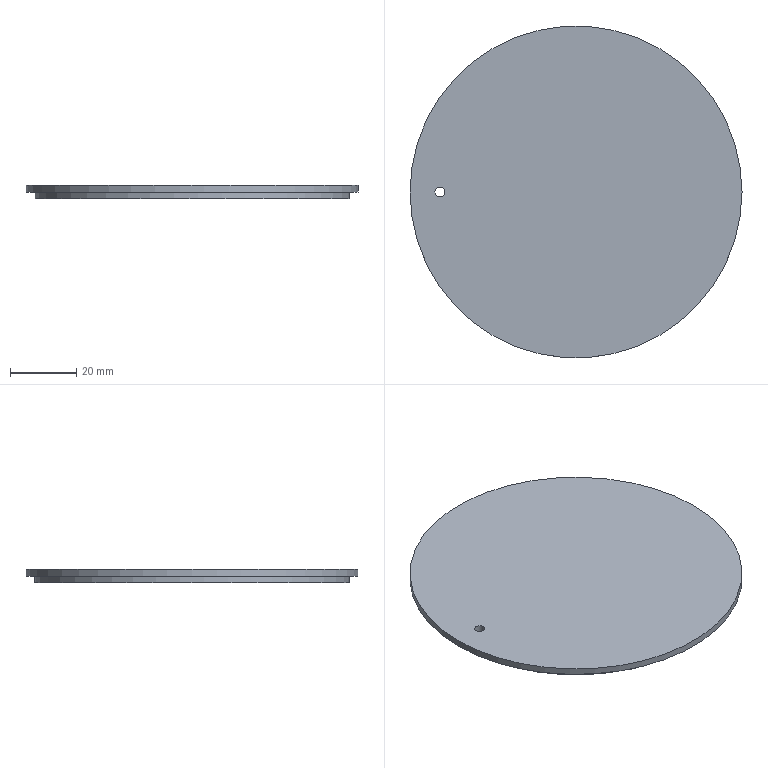Component | NX | BASE_COVER | 1 solid | 6 faces | box 100 x 100 x 4 mm | volume 29796 mm3 | cylinder 3 | plane 3 | commonest cylinder face diameters 94.8 x1 100 x1 3 x1
STEP:
#1=CARTESIAN_POINT('',(0.,0.,0.));
#2=DIRECTION('',(0.,0.,1.));
#3=DIRECTION('',(1.,0.,0.));
#4=AXIS2_PLACEMENT_3D('',#1,#2,#3);
#5=CARTESIAN_POINT('',(45.896,-15.585,-0.4905));
#6=VERTEX_POINT('',#5);
#7=CARTESIAN_POINT('',(-1.504,-15.585,-0.4905));
#8=DIRECTION('',(0.,0.,-1.));
#9=DIRECTION('',(1.,0.,0.));
#10=AXIS2_PLACEMENT_3D('',#7,#8,#9);
#11=CIRCLE('',#10,47.4);
#12=CARTESIAN_POINT('',(-1.504,-15.585,-0.4905));
#13=DIRECTION('',(0.,0.,-1.));
#14=DIRECTION('',(1.,0.,0.));
#15=AXIS2_PLACEMENT_3D('',#12,#13,#14);
#16=CYLINDRICAL_SURFACE('',#15,47.4);
#17=CARTESIAN_POINT('',(0.,0.));
#18=DIRECTION('',(1.,0.));
#19=VECTOR('',#18,1.);
#20=LINE('',#17,#19);
#21=(GEOMETRIC_REPRESENTATION_CONTEXT(2)PARAMETRIC_REPRESENTATION_CONTEXT()REPRESENTATION_CONTEXT('',''));
#22=DEFINITIONAL_REPRESENTATION('',(#20),#21);
#23=PCURVE('',#16,#22);
#24=CARTESIAN_POINT('',(-1.504,-15.585,-0.4905));
#25=DIRECTION('',(0.,0.,-1.));
#26=DIRECTION('',(1.,0.,0.));
#27=AXIS2_PLACEMENT_3D('',#24,#25,#26);
#28=PLANE('',#27);
#29=CARTESIAN_POINT('',(0.,0.));
#30=DIRECTION('',(1.,0.));
#31=AXIS2_PLACEMENT_2D('',#29,#30);
#32=CIRCLE('',#31,47.4);
#33=(GEOMETRIC_REPRESENTATION_CONTEXT(2)PARAMETRIC_REPRESENTATION_CONTEXT()REPRESENTATION_CONTEXT('',''));
#34=DEFINITIONAL_REPRESENTATION('',(#32),#33);
#35=PCURVE('',#28,#34);
#36=SURFACE_CURVE('',#11,(#23,#35),.PCURVE_S1.);
#37=EDGE_CURVE('',#6,#6,#36,.T.);
#38=ORIENTED_EDGE('',*,*,#37,.T.);
#39=CARTESIAN_POINT('',(45.896,-15.585,-2.49));
#40=VERTEX_POINT('',#39);
#41=CARTESIAN_POINT('',(45.896,-15.585,-0.4905));
#42=CARTESIAN_POINT('',(45.896,-15.585,-2.49));
#43=B_SPLINE_CURVE_WITH_KNOTS('',1,(#41,#42),.UNSPECIFIED.,.F.,.F.,(2,2),(0.,2.),.PIECEWISE_BEZIER_KNOTS.);
#44=CARTESIAN_POINT('',(6.283,0.));
#45=DIRECTION('',(0.,1.));
#46=VECTOR('',#45,1.);
#47=LINE('',#44,#46);
#48=(GEOMETRIC_REPRESENTATION_CONTEXT(2)PARAMETRIC_REPRESENTATION_CONTEXT()REPRESENTATION_CONTEXT('',''));
#49=DEFINITIONAL_REPRESENTATION('',(#47),#48);
#50=PCURVE('',#16,#49);
#51=CARTESIAN_POINT('',(0.,0.));
#52=DIRECTION('',(0.,1.));
#53=VECTOR('',#52,1.);
#54=LINE('',#51,#53);
#55=(GEOMETRIC_REPRESENTATION_CONTEXT(2)PARAMETRIC_REPRESENTATION_CONTEXT()REPRESENTATION_CONTEXT('',''));
#56=DEFINITIONAL_REPRESENTATION('',(#54),#55);
#57=PCURVE('',#16,#56);
#58=SEAM_CURVE('',#43,(#50,#57),.PCURVE_S1.);
#59=EDGE_CURVE('',#6,#40,#58,.T.);
#60=ORIENTED_EDGE('',*,*,#59,.T.);
#61=CARTESIAN_POINT('',(-1.504,-15.585,-2.49));
#62=DIRECTION('',(0.,0.,-1.));
#63=DIRECTION('',(1.,0.,0.));
#64=AXIS2_PLACEMENT_3D('',#61,#62,#63);
#65=CIRCLE('',#64,47.4);
#66=CARTESIAN_POINT('',(0.,2.));
#67=DIRECTION('',(1.,0.));
#68=VECTOR('',#67,1.);
#69=LINE('',#66,#68);
#70=(GEOMETRIC_REPRESENTATION_CONTEXT(2)PARAMETRIC_REPRESENTATION_CONTEXT()REPRESENTATION_CONTEXT('',''));
#71=DEFINITIONAL_REPRESENTATION('',(#69),#70);
#72=PCURVE('',#16,#71);
#73=CARTESIAN_POINT('',(-1.504,-15.585,-2.49));
#74=DIRECTION('',(0.,0.,-1.));
#75=DIRECTION('',(1.,0.,0.));
#76=AXIS2_PLACEMENT_3D('',#73,#74,#75);
#77=PLANE('',#76);
#78=CARTESIAN_POINT('',(0.,0.));
#79=DIRECTION('',(1.,0.));
#80=AXIS2_PLACEMENT_2D('',#78,#79);
#81=CIRCLE('',#80,47.4);
#82=(GEOMETRIC_REPRESENTATION_CONTEXT(2)PARAMETRIC_REPRESENTATION_CONTEXT()REPRESENTATION_CONTEXT('',''));
#83=DEFINITIONAL_REPRESENTATION('',(#81),#82);
#84=PCURVE('',#77,#83);
#85=SURFACE_CURVE('',#65,(#72,#84),.PCURVE_S1.);
#86=EDGE_CURVE('',#40,#40,#85,.T.);
#87=ORIENTED_EDGE('',*,*,#86,.F.);
#88=ORIENTED_EDGE('',*,*,#59,.F.);
#89=EDGE_LOOP('',(#38,#60,#87,#88));
#90=FACE_BOUND('',#89,.T.);
#91=ADVANCED_FACE('',(#90),#16,.T.);
#92=CARTESIAN_POINT('',(-41.004,-15.585,-2.49));
#93=VERTEX_POINT('',#92);
#94=CARTESIAN_POINT('',(-42.504,-15.585,-2.49));
#95=DIRECTION('',(0.,0.,-1.));
#96=DIRECTION('',(1.,0.,0.));
#97=AXIS2_PLACEMENT_3D('',#94,#95,#96);
#98=CIRCLE('',#97,1.5);
#99=CARTESIAN_POINT('',(-41.,0.));
#100=DIRECTION('',(1.,0.));
#101=AXIS2_PLACEMENT_2D('',#99,#100);
#102=CIRCLE('',#101,1.5);
#103=(GEOMETRIC_REPRESENTATION_CONTEXT(2)PARAMETRIC_REPRESENTATION_CONTEXT()REPRESENTATION_CONTEXT('',''));
#104=DEFINITIONAL_REPRESENTATION('',(#102),#103);
#105=PCURVE('',#77,#104);
#106=CARTESIAN_POINT('',(-42.504,-15.585,8.01));
#107=DIRECTION('',(0.,0.,-1.));
#108=DIRECTION('',(1.,0.,0.));
#109=AXIS2_PLACEMENT_3D('',#106,#107,#108);
#110=CYLINDRICAL_SURFACE('',#109,1.5);
#111=CARTESIAN_POINT('',(0.,10.5));
#112=DIRECTION('',(1.,0.));
#113=VECTOR('',#112,1.);
#114=LINE('',#111,#113);
#115=(GEOMETRIC_REPRESENTATION_CONTEXT(2)PARAMETRIC_REPRESENTATION_CONTEXT()REPRESENTATION_CONTEXT('',''));
#116=DEFINITIONAL_REPRESENTATION('',(#114),#115);
#117=PCURVE('',#110,#116);
#118=SURFACE_CURVE('',#98,(#105,#117),.PCURVE_S1.);
#119=EDGE_CURVE('',#93,#93,#118,.T.);
#120=ORIENTED_EDGE('',*,*,#119,.F.);
#121=EDGE_LOOP('',(#120));
#122=FACE_BOUND('',#121,.T.);
#123=ORIENTED_EDGE('',*,*,#86,.T.);
#124=EDGE_LOOP('',(#123));
#125=FACE_BOUND('',#124,.T.);
#126=ADVANCED_FACE('',(#122,#125),#77,.T.);
#127=CARTESIAN_POINT('',(48.496,-15.585,-0.4905));
#128=VERTEX_POINT('',#127);
#129=CARTESIAN_POINT('',(-1.504,-15.585,-0.4905));
#130=DIRECTION('',(0.,0.,-1.));
#131=DIRECTION('',(1.,0.,0.));
#132=AXIS2_PLACEMENT_3D('',#129,#130,#131);
#133=CIRCLE('',#132,50.);
#134=CARTESIAN_POINT('',(-1.504,-15.585,-0.4905));
#135=DIRECTION('',(0.,0.,1.));
#136=DIRECTION('',(-1.,0.,0.));
#137=AXIS2_PLACEMENT_3D('',#134,#135,#136);
#138=CYLINDRICAL_SURFACE('',#137,50.);
#139=CARTESIAN_POINT('',(9.425,0.));
#140=DIRECTION('',(-1.,0.));
#141=VECTOR('',#140,1.);
#142=LINE('',#139,#141);
#143=(GEOMETRIC_REPRESENTATION_CONTEXT(2)PARAMETRIC_REPRESENTATION_CONTEXT()REPRESENTATION_CONTEXT('',''));
#144=DEFINITIONAL_REPRESENTATION('',(#142),#143);
#145=PCURVE('',#138,#144);
#146=CARTESIAN_POINT('',(0.,0.));
#147=DIRECTION('',(1.,0.));
#148=AXIS2_PLACEMENT_2D('',#146,#147);
#149=CIRCLE('',#148,50.);
#150=(GEOMETRIC_REPRESENTATION_CONTEXT(2)PARAMETRIC_REPRESENTATION_CONTEXT()REPRESENTATION_CONTEXT('',''));
#151=DEFINITIONAL_REPRESENTATION('',(#149),#150);
#152=PCURVE('',#28,#151);
#153=SURFACE_CURVE('',#133,(#145,#152),.PCURVE_S1.);
#154=EDGE_CURVE('',#128,#128,#153,.T.);
#155=ORIENTED_EDGE('',*,*,#154,.F.);
#156=CARTESIAN_POINT('',(48.496,-15.585,1.51));
#157=VERTEX_POINT('',#156);
#158=CARTESIAN_POINT('',(48.496,-15.585,-0.4905));
#159=CARTESIAN_POINT('',(48.496,-15.585,1.51));
#160=B_SPLINE_CURVE_WITH_KNOTS('',1,(#158,#159),.UNSPECIFIED.,.F.,.F.,(2,2),(0.,2.),.PIECEWISE_BEZIER_KNOTS.);
#161=CARTESIAN_POINT('',(9.425,0.));
#162=DIRECTION('',(0.,1.));
#163=VECTOR('',#162,1.);
#164=LINE('',#161,#163);
#165=(GEOMETRIC_REPRESENTATION_CONTEXT(2)PARAMETRIC_REPRESENTATION_CONTEXT()REPRESENTATION_CONTEXT('',''));
#166=DEFINITIONAL_REPRESENTATION('',(#164),#165);
#167=PCURVE('',#138,#166);
#168=CARTESIAN_POINT('',(3.142,0.));
#169=DIRECTION('',(0.,1.));
#170=VECTOR('',#169,1.);
#171=LINE('',#168,#170);
#172=(GEOMETRIC_REPRESENTATION_CONTEXT(2)PARAMETRIC_REPRESENTATION_CONTEXT()REPRESENTATION_CONTEXT('',''));
#173=DEFINITIONAL_REPRESENTATION('',(#171),#172);
#174=PCURVE('',#138,#173);
#175=SEAM_CURVE('',#160,(#167,#174),.PCURVE_S1.);
#176=EDGE_CURVE('',#128,#157,#175,.T.);
#177=ORIENTED_EDGE('',*,*,#176,.T.);
#178=CARTESIAN_POINT('',(-1.504,-15.585,1.51));
#179=DIRECTION('',(0.,0.,-1.));
#180=DIRECTION('',(1.,0.,0.));
#181=AXIS2_PLACEMENT_3D('',#178,#179,#180);
#182=CIRCLE('',#181,50.);
#183=CARTESIAN_POINT('',(9.425,2.));
#184=DIRECTION('',(-1.,0.));
#185=VECTOR('',#184,1.);
#186=LINE('',#183,#185);
#187=(GEOMETRIC_REPRESENTATION_CONTEXT(2)PARAMETRIC_REPRESENTATION_CONTEXT()REPRESENTATION_CONTEXT('',''));
#188=DEFINITIONAL_REPRESENTATION('',(#186),#187);
#189=PCURVE('',#138,#188);
#190=CARTESIAN_POINT('',(-1.504,-15.585,1.51));
#191=DIRECTION('',(0.,0.,-1.));
#192=DIRECTION('',(1.,0.,0.));
#193=AXIS2_PLACEMENT_3D('',#190,#191,#192);
#194=PLANE('',#193);
#195=CARTESIAN_POINT('',(0.,0.));
#196=DIRECTION('',(1.,0.));
#197=AXIS2_PLACEMENT_2D('',#195,#196);
#198=CIRCLE('',#197,50.);
#199=(GEOMETRIC_REPRESENTATION_CONTEXT(2)PARAMETRIC_REPRESENTATION_CONTEXT()REPRESENTATION_CONTEXT('',''));
#200=DEFINITIONAL_REPRESENTATION('',(#198),#199);
#201=PCURVE('',#194,#200);
#202=SURFACE_CURVE('',#182,(#189,#201),.PCURVE_S1.);
#203=EDGE_CURVE('',#157,#157,#202,.T.);
#204=ORIENTED_EDGE('',*,*,#203,.T.);
#205=ORIENTED_EDGE('',*,*,#176,.F.);
#206=EDGE_LOOP('',(#155,#177,#204,#205));
#207=FACE_BOUND('',#206,.T.);
#208=ADVANCED_FACE('',(#207),#138,.T.);
#209=ORIENTED_EDGE('',*,*,#37,.F.);
#210=EDGE_LOOP('',(#209));
#211=FACE_BOUND('',#210,.T.);
#212=ORIENTED_EDGE('',*,*,#154,.T.);
#213=EDGE_LOOP('',(#212));
#214=FACE_BOUND('',#213,.T.);
#215=ADVANCED_FACE('',(#211,#214),#28,.T.);
#216=CARTESIAN_POINT('',(-41.004,-15.585,1.51));
#217=VERTEX_POINT('',#216);
#218=CARTESIAN_POINT('',(-42.504,-15.585,1.51));
#219=DIRECTION('',(0.,0.,-1.));
#220=DIRECTION('',(1.,0.,0.));
#221=AXIS2_PLACEMENT_3D('',#218,#219,#220);
#222=CIRCLE('',#221,1.5);
#223=CARTESIAN_POINT('',(-41.,0.));
#224=DIRECTION('',(1.,0.));
#225=AXIS2_PLACEMENT_2D('',#223,#224);
#226=CIRCLE('',#225,1.5);
#227=(GEOMETRIC_REPRESENTATION_CONTEXT(2)PARAMETRIC_REPRESENTATION_CONTEXT()REPRESENTATION_CONTEXT('',''));
#228=DEFINITIONAL_REPRESENTATION('',(#226),#227);
#229=PCURVE('',#194,#228);
#230=CARTESIAN_POINT('',(0.,6.5));
#231=DIRECTION('',(1.,0.));
#232=VECTOR('',#231,1.);
#233=LINE('',#230,#232);
#234=(GEOMETRIC_REPRESENTATION_CONTEXT(2)PARAMETRIC_REPRESENTATION_CONTEXT()REPRESENTATION_CONTEXT('',''));
#235=DEFINITIONAL_REPRESENTATION('',(#233),#234);
#236=PCURVE('',#110,#235);
#237=SURFACE_CURVE('',#222,(#229,#236),.PCURVE_S1.);
#238=EDGE_CURVE('',#217,#217,#237,.T.);
#239=ORIENTED_EDGE('',*,*,#238,.T.);
#240=EDGE_LOOP('',(#239));
#241=FACE_BOUND('',#240,.T.);
#242=ORIENTED_EDGE('',*,*,#203,.F.);
#243=EDGE_LOOP('',(#242));
#244=FACE_BOUND('',#243,.T.);
#245=ADVANCED_FACE('',(#241,#244),#194,.F.);
#246=ORIENTED_EDGE('',*,*,#119,.F.);
#247=CARTESIAN_POINT('',(-41.004,-15.585,1.51));
#248=CARTESIAN_POINT('',(-41.004,-15.585,-2.49));
#249=B_SPLINE_CURVE_WITH_KNOTS('',1,(#247,#248),.UNSPECIFIED.,.F.,.F.,(2,2),(6.5,10.5),.PIECEWISE_BEZIER_KNOTS.);
#250=CARTESIAN_POINT('',(0.,0.));
#251=DIRECTION('',(0.,1.));
#252=VECTOR('',#251,1.);
#253=LINE('',#250,#252);
#254=(GEOMETRIC_REPRESENTATION_CONTEXT(2)PARAMETRIC_REPRESENTATION_CONTEXT()REPRESENTATION_CONTEXT('',''));
#255=DEFINITIONAL_REPRESENTATION('',(#253),#254);
#256=PCURVE('',#110,#255);
#257=CARTESIAN_POINT('',(6.283,0.));
#258=DIRECTION('',(0.,1.));
#259=VECTOR('',#258,1.);
#260=LINE('',#257,#259);
#261=(GEOMETRIC_REPRESENTATION_CONTEXT(2)PARAMETRIC_REPRESENTATION_CONTEXT()REPRESENTATION_CONTEXT('',''));
#262=DEFINITIONAL_REPRESENTATION('',(#260),#261);
#263=PCURVE('',#110,#262);
#264=SEAM_CURVE('',#249,(#256,#263),.PCURVE_S1.);
#265=EDGE_CURVE('',#217,#93,#264,.T.);
#266=ORIENTED_EDGE('',*,*,#265,.F.);
#267=ORIENTED_EDGE('',*,*,#238,.T.);
#268=ORIENTED_EDGE('',*,*,#265,.T.);
#269=EDGE_LOOP('',(#246,#266,#267,#268));
#270=FACE_BOUND('',#269,.F.);
#271=ADVANCED_FACE('',(#270),#110,.F.);
#272=CLOSED_SHELL('',(#91,#126,#208,#215,#245,#271));
#273=MANIFOLD_SOLID_BREP('',#272);
#274=(LENGTH_UNIT()NAMED_UNIT(*)SI_UNIT(.MILLI.,.METRE.));
#275=UNCERTAINTY_MEASURE_WITH_UNIT(LENGTH_MEASURE(0.00001),#274,'','');
#276=(NAMED_UNIT(*)PLANE_ANGLE_UNIT()SI_UNIT($,.RADIAN.));
#277=(NAMED_UNIT(*)SI_UNIT($,.STERADIAN.)SOLID_ANGLE_UNIT());
#278=(GEOMETRIC_REPRESENTATION_CONTEXT(3)GLOBAL_UNCERTAINTY_ASSIGNED_CONTEXT((#275))GLOBAL_UNIT_ASSIGNED_CONTEXT((#274,#276,#277))REPRESENTATION_CONTEXT('',''));
#279=ADVANCED_BREP_SHAPE_REPRESENTATION('',(#4,#273),#278);